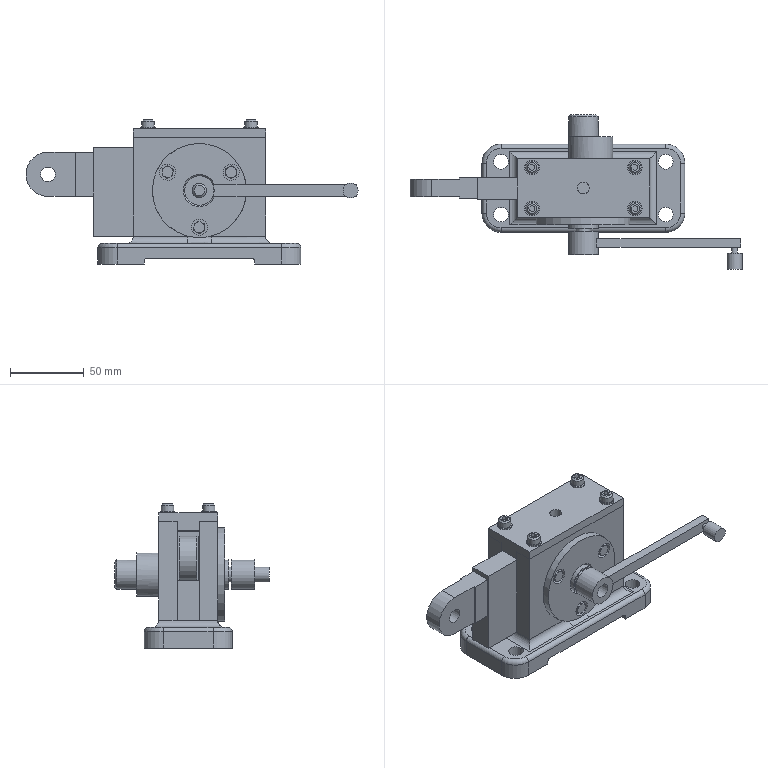Assembly | NX | mm | 18 component files | 18 solids | 271 faces | box 225.95 x 105.27 x 98 mm | volume 415290 mm3 | plane 154 | cylinder 76 | cone 36 | torus 4 | spline 1 | commonest cylinder face diameters 10 x17 5 x14 6 x8 5.5 x7 20 x6 26 x4 8.5 x4 4 x3
Bill of materials:
unnamed part 1 | 1 |  | Thin-walled cylindrical ring or sleeve: a short open tube whose axial length is noticeably greater than its wall thickness.
unnamed part 2 | 3 |  | Hex-head, bolt-like part: a hexagonal head with chamfered corners on one face, joined to a plain cylindrical shank with a chamfered tip.
unnamed part 3 | 1 |  | Round flange with a raised cylindrical hub on one side, a central through bore, and three smaller through holes on a bolt circle.
unnamed part 4 | 4 |  | Socket-head, cap-screw-like part: a cylindrical head with a hexagonal socket recess and a chamfered top edge, on a plain cylindrical shank with a chamfered end.
unnamed part 5 | 1 |  | Flat plate-like link: a narrower tongue with a rounded end and a small round through hole, joined to a wider rectangular body that has a rectangular through window.
unnamed part 6 | 1 |  | Rectangular flat plate with four corner through holes and one larger central through hole, plus a rectangular key- or rib-like block protruding from the underside.
unnamed part 7 | 4 |  | Flat annular disc shaped like a plain washer: a thin ring with a large central hole.
unnamed part 8 | 1 |  | Crank- or lever-like arm: a cylindrical boss with a through bore at one end, a straight rectangular-section bar, and a small cylindrical pin at the far end. The pin has a reduced neck and is offset perpendicular to the bar.
unnamed part 9 | 1 |  | Bracket or pedestal-style support: a rounded-rectangle base with four corner through holes, carrying two parallel upright plates with a gap between them. The uprights have a central through hole, a circular recessed pocket with small holes on one face, and small holes in their top edges.
unnamed part 10 | 1 |  | Stepped, shaft-like pin: a small-diameter end pin with a chamfered end, a tapered section, a cylindrical main section, an eccentric (off-centre) cylindrical collar, and a short chamfered end journal.
Mates:
1. concentric | upper_cover 1 edge | housing 1 edge
2. parallel | upper_cover 1 face | housing 1 face
3. align lock | eccentric_shaft 1 face | housing 1 face
4. touch align | eccentric_shaft 1 face | housing 1 face
5. concentric | washer 4 edge | upper_cover 1 edge
6. concentric | hex_socket_screw 4 edge | washer 4 edge
7. bond | upper_cover 1 component | assembly component
8. bond | hex_socket_screw 4 component | assembly component
9. bond | washer 4 component | assembly component
10. bond | hex_socket_screw 3 component | assembly component
11. bond | washer 3 component | assembly component
12. linear | assembly datumaxis | assembly cartesiancoordinatesystem | assembly cartesiancoordinatesystem
13. linear | assembly datumaxis | assembly cartesiancoordinatesystem | assembly cartesiancoordinatesystem
14. fix | assembly component
15. bond | hex_socket_screw 4 component | assembly component
16. bond | washer 4 component | assembly component
17. bond | washer 3 component | assembly component
18. bond | hex_socket_screw 3 component | assembly component
19. bond | hex_socket_screw 2 component | assembly component
20. bond | washer 2 component | assembly component
21. bond | washer 1 component | assembly component
22. bond | hex_socket_screw 1 component | assembly component
23. linear | assembly datumaxis | assembly cartesiancoordinatesystem | assembly cartesiancoordinatesystem
24. linear | assembly datumaxis | assembly cartesiancoordinatesystem | assembly cartesiancoordinatesystem
25. linear | assembly datumaxis | assembly cartesiancoordinatesystem | assembly cartesiancoordinatesystem
26. linear | assembly datumaxis | assembly cartesiancoordinatesystem | assembly cartesiancoordinatesystem
27. parallel | push_rod 1 face | housing 1 face
28. parallel | push_rod 1 face | housing 1 face
29. touch align | push_rod 1 face | housing 1 face
30. touch align | push_rod 1 face | housing 1 edge
31. align lock | flange_cover 1 face | housing 1 face
32. touch align | flange_cover 1 edge | housing 1 face
33. concentric | hex_screw 3 edge | flange_cover 1 edge
34. fix | assembly component
35. bond | hex_screw 3 component | assembly component
36. bond | hex_screw 2 component | assembly component
37. bond | hex_screw 1 component | assembly component
38. circular | assembly datumaxis | assembly cartesiancoordinatesystem | assembly cartesiancoordinatesystem | assembly cartesiancoordinatesystem